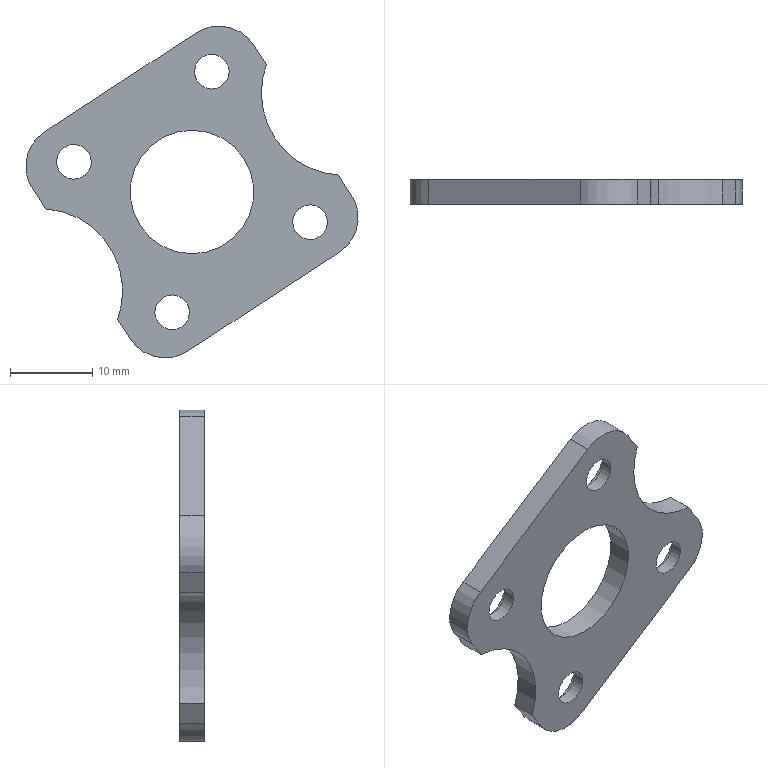Component | SolidWorks | FrontWheelBearingPlate-2 | 1 solid | 37 faces | box 40.34 x 3 x 40.28 mm | volume 1835 mm3 | cylinder 25 | plane 12 | commonest cylinder face diameters 7.6 x8 4.2 x8 10 x4 20 x3 15 x2
build123d program:
from build123d import *

# Parameters (mm, degrees)
SKETCH1_W           = 32
SKETCH1_H           = 31.8
SKETCH1_R           = 2.1
SKETCH1_R_2         = 7.5
BOSS_EXTRUDE1_DEPTH = 3
SKETCH2_R           = 10
CUT_EXTRUDE1_DEPTH  = 23.755
FILLET1_R           = 5
SKETCH3_R           = 3.8
CUT_EXTRUDE2_DEPTH  = 1.5


with BuildPart() as part:
    # Sketch1 → Boss-Extrude1 (new body)
    with BuildSketch(Plane.XY):
        Rectangle(SKETCH1_W, SKETCH1_H)
        with Locations((-10, 10.9)):
            Circle(SKETCH1_R, mode=Mode.SUBTRACT)
        with Locations(Location((10, 10.9, 0), (0, 0, 180))):
            Circle(SKETCH1_R, mode=Mode.SUBTRACT)
        with Locations((10, -10.9)):
            Circle(SKETCH1_R, mode=Mode.SUBTRACT)
        with Locations(Location((-10, -10.9, 0), (0, 0, 180))):
            Circle(SKETCH1_R, mode=Mode.SUBTRACT)
        Circle(SKETCH1_R_2, mode=Mode.SUBTRACT)
    extrude(amount=BOSS_EXTRUDE1_DEPTH)

    # Sketch2 → Cut-Extrude1 (cut, through all)
    with BuildSketch(Plane.XY.offset(3)):
        with Locations((22, 0)):
            Circle(SKETCH2_R)
        with Locations((-22, 0)):
            Circle(SKETCH2_R)
    extrude(amount=-CUT_EXTRUDE1_DEPTH, mode=Mode.SUBTRACT)

    # Fillet1
    fillet1_edges = [part.edges().sort_by_distance(p)[0] for p in [
        (16, -15.9, 1.5),
        (-16, -15.9, 1.5),
        (-16, 15.9, 1.5),
        (16, 15.9, 1.5),
    ]]
    fillet(fillet1_edges, radius=FILLET1_R)

    # Sketch3 → Cut-Extrude2 (cut)
    with BuildSketch(Plane.XY.offset(3)):
        with Locations((-10, 10.9)):
            Circle(SKETCH3_R)
        with Locations((10, 10.9)):
            Circle(SKETCH3_R)
        with Locations((10, -10.9)):
            Circle(SKETCH3_R)
        with Locations((-10, -10.9)):
            Circle(SKETCH3_R)
    extrude(amount=-CUT_EXTRUDE2_DEPTH, mode=Mode.SUBTRACT)


solid = part.part

# Placed as in the assembly
solid = solid.moved(Location((0.3183, -13.6, 37), (-90, 0, 146.842)))